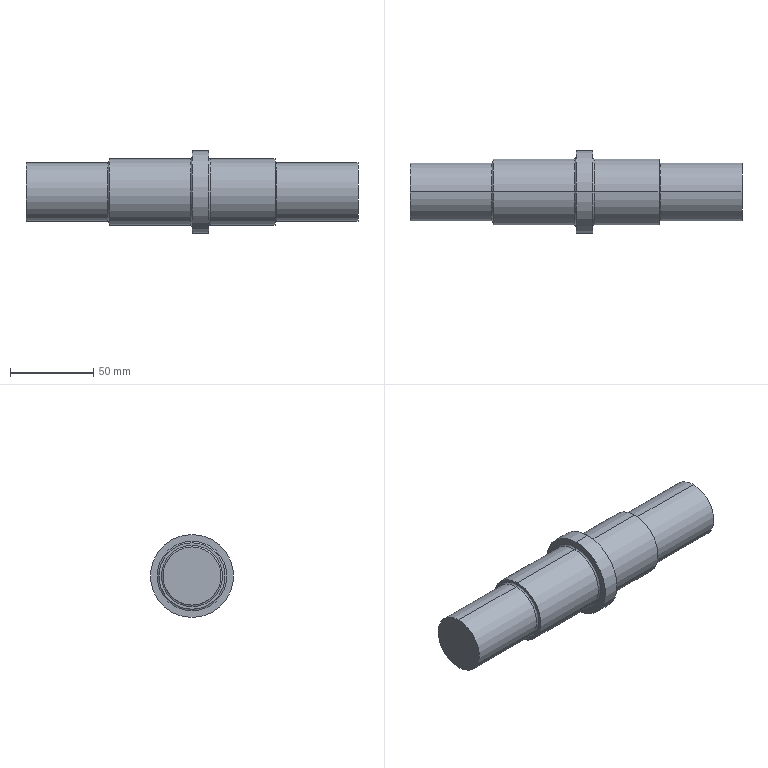Component | SolidWorks | AxisTwo-1 | 1 solid | 24 faces | box 200 x 50 x 50 mm | volume 229046 mm3 | cylinder 10 | torus 8 | plane 6 | commonest cylinder face diameters 35 x4 40 x4 50 x2
build123d program:
from build123d import *


with BuildPart() as part:
    # Sketch1 → Revolve1 (revolve)
    with BuildSketch(Plane(origin=(0, 0, 0), x_dir=(0, 0, -1), z_dir=(1, 0, 0)), mode=Mode.PRIVATE) as revolve1_sk:
        with BuildLine():
            Line((0, 0), (0, 17.5))
            Line((0, 17.5), (49, 17.5))
            ThreePointArc((49, 17.5), (49.707, 17.793), (50, 18.5))
            Line((50, 18.5), (50, 20))
            Line((50, 20), (89, 20))
            ThreePointArc((89, 20), (89.707, 20.293), (90, 21))
            Line((90, 21), (90, 25))
            Line((90, 25), (100, 25))
            Line((100, 25), (100, 21))
            ThreePointArc((100, 21), (100.293, 20.293), (101, 20))
            Line((101, 20), (150, 20))
            Line((150, 20), (150, 18.5))
            ThreePointArc((150, 18.5), (150.293, 17.793), (151, 17.5))
            Line((151, 17.5), (200, 17.5))
            Line((200, 17.5), (200, 0))
            Line((200, 0), (0, 0))
        make_face()
    revolve(revolve1_sk.sketch.rotate(Axis((0, 0, -200), (0, 0, 1)), 90), axis=Axis((0, 0, -200), (0, 0, 1)))


solid = part.part

# Placed as in the assembly
solid = solid.moved(Location((300.528, 15.31, -110), (0, 90, 0)))
STEP:
#1=COLOUR_RGB('',0.7922,0.8196,0.9333);
#2=FILL_AREA_STYLE_COLOUR('',#1);
#3=FILL_AREA_STYLE('',(#2));
#4=SURFACE_STYLE_FILL_AREA(#3);
#5=SURFACE_SIDE_STYLE('',(#4));
#6=SURFACE_STYLE_USAGE(.BOTH.,#5);
#7=PRESENTATION_STYLE_ASSIGNMENT((#6));
#8=CARTESIAN_POINT('',(11.832,0.6028,-3.642));
#9=VERTEX_POINT('',#8);
#10=CARTESIAN_POINT('',(11.832,0.6028,-5.02));
#11=VERTEX_POINT('',#10);
#12=CARTESIAN_POINT('',(11.832,0.6028,-4.331));
#13=DIRECTION('',(-1.,0.,0.));
#14=DIRECTION('',(0.,0.,1.));
#15=AXIS2_PLACEMENT_3D('',#12,#13,#14);
#16=CIRCLE('',#15,0.689);
#17=EDGE_CURVE('',#9,#11,#16,.T.);
#18=ORIENTED_EDGE('',*,*,#17,.T.);
#19=CARTESIAN_POINT('',(9.903,0.6028,-5.02));
#20=VERTEX_POINT('',#19);
#21=CARTESIAN_POINT('',(3.958,0.6028,-5.02));
#22=DIRECTION('',(-1.,0.,0.));
#23=VECTOR('',#22,39.37);
#24=LINE('',#21,#23);
#25=EDGE_CURVE('',#11,#20,#24,.T.);
#26=ORIENTED_EDGE('',*,*,#25,.T.);
#27=CARTESIAN_POINT('',(9.903,0.6028,-3.642));
#28=VERTEX_POINT('',#27);
#29=CARTESIAN_POINT('',(9.903,0.6028,-4.331));
#30=DIRECTION('',(-1.,0.,0.));
#31=DIRECTION('',(0.,0.,1.));
#32=AXIS2_PLACEMENT_3D('',#29,#30,#31);
#33=CIRCLE('',#32,0.689);
#34=EDGE_CURVE('',#28,#20,#33,.T.);
#35=ORIENTED_EDGE('',*,*,#34,.F.);
#36=CARTESIAN_POINT('',(3.958,0.6028,-3.642));
#37=DIRECTION('',(-1.,0.,0.));
#38=VECTOR('',#37,39.37);
#39=LINE('',#36,#38);
#40=EDGE_CURVE('',#9,#28,#39,.T.);
#41=ORIENTED_EDGE('',*,*,#40,.F.);
#42=EDGE_LOOP('',(#18,#26,#35,#41));
#43=FACE_OUTER_BOUND('',#42,.T.);
#44=CARTESIAN_POINT('',(3.958,0.6028,-4.331));
#45=DIRECTION('',(-1.,0.,0.));
#46=DIRECTION('',(0.,0.,1.));
#47=AXIS2_PLACEMENT_3D('',#44,#45,#46);
#48=CYLINDRICAL_SURFACE('',#47,0.689);
#49=ADVANCED_FACE('',(#43),#48,.T.);
#50=CARTESIAN_POINT('',(9.863,0.6028,-5.059));
#51=VERTEX_POINT('',#50);
#52=CARTESIAN_POINT('',(9.863,0.6028,-3.602));
#53=VERTEX_POINT('',#52);
#54=CARTESIAN_POINT('',(9.863,0.6028,-4.331));
#55=DIRECTION('',(-1.,0.,0.));
#56=DIRECTION('',(0.,0.,1.));
#57=AXIS2_PLACEMENT_3D('',#54,#55,#56);
#58=CIRCLE('',#57,0.7283);
#59=EDGE_CURVE('',#51,#53,#58,.T.);
#60=ORIENTED_EDGE('',*,*,#59,.F.);
#61=CARTESIAN_POINT('',(9.903,0.6028,-5.059));
#62=DIRECTION('',(0.,1.,0.));
#63=DIRECTION('',(0.,0.,1.));
#64=AXIS2_PLACEMENT_3D('',#61,#62,#63);
#65=CIRCLE('',#64,0.03937);
#66=EDGE_CURVE('',#51,#20,#65,.T.);
#67=ORIENTED_EDGE('',*,*,#66,.T.);
#68=CARTESIAN_POINT('',(9.903,0.6028,-4.331));
#69=DIRECTION('',(-1.,0.,0.));
#70=DIRECTION('',(0.,0.,1.));
#71=AXIS2_PLACEMENT_3D('',#68,#69,#70);
#72=CIRCLE('',#71,0.689);
#73=EDGE_CURVE('',#20,#28,#72,.T.);
#74=ORIENTED_EDGE('',*,*,#73,.T.);
#75=CARTESIAN_POINT('',(9.903,0.6028,-3.602));
#76=DIRECTION('',(0.,-1.,0.));
#77=DIRECTION('',(0.,0.,-1.));
#78=AXIS2_PLACEMENT_3D('',#75,#76,#77);
#79=CIRCLE('',#78,0.03937);
#80=EDGE_CURVE('',#53,#28,#79,.T.);
#81=ORIENTED_EDGE('',*,*,#80,.F.);
#82=EDGE_LOOP('',(#60,#67,#74,#81));
#83=FACE_OUTER_BOUND('',#82,.T.);
#84=CARTESIAN_POINT('',(9.903,0.6028,-4.331));
#85=DIRECTION('',(-1.,0.,0.));
#86=DIRECTION('',(0.,0.,1.));
#87=AXIS2_PLACEMENT_3D('',#84,#85,#86);
#88=TOROIDAL_SURFACE('',#87,0.7283,0.03937);
#89=ADVANCED_FACE('',(#83),#88,.F.);
#90=CARTESIAN_POINT('',(9.863,0.6028,-3.543));
#91=VERTEX_POINT('',#90);
#92=CARTESIAN_POINT('',(9.863,0.6028,-5.118));
#93=VERTEX_POINT('',#92);
#94=CARTESIAN_POINT('',(9.863,0.6028,-4.331));
#95=DIRECTION('',(-1.,0.,0.));
#96=DIRECTION('',(0.,0.,1.));
#97=AXIS2_PLACEMENT_3D('',#94,#95,#96);
#98=CIRCLE('',#97,0.7874);
#99=EDGE_CURVE('',#91,#93,#98,.T.);
#100=ORIENTED_EDGE('',*,*,#99,.T.);
#101=CARTESIAN_POINT('',(8.328,0.6028,-5.118));
#102=VERTEX_POINT('',#101);
#103=CARTESIAN_POINT('',(3.958,0.6028,-5.118));
#104=DIRECTION('',(-1.,0.,0.));
#105=VECTOR('',#104,39.37);
#106=LINE('',#103,#105);
#107=EDGE_CURVE('',#93,#102,#106,.T.);
#108=ORIENTED_EDGE('',*,*,#107,.T.);
#109=CARTESIAN_POINT('',(8.328,0.6028,-3.543));
#110=VERTEX_POINT('',#109);
#111=CARTESIAN_POINT('',(8.328,0.6028,-4.331));
#112=DIRECTION('',(-1.,0.,0.));
#113=DIRECTION('',(0.,0.,1.));
#114=AXIS2_PLACEMENT_3D('',#111,#112,#113);
#115=CIRCLE('',#114,0.7874);
#116=EDGE_CURVE('',#110,#102,#115,.T.);
#117=ORIENTED_EDGE('',*,*,#116,.F.);
#118=CARTESIAN_POINT('',(3.958,0.6028,-3.543));
#119=DIRECTION('',(-1.,0.,0.));
#120=VECTOR('',#119,39.37);
#121=LINE('',#118,#120);
#122=EDGE_CURVE('',#91,#110,#121,.T.);
#123=ORIENTED_EDGE('',*,*,#122,.F.);
#124=EDGE_LOOP('',(#100,#108,#117,#123));
#125=FACE_OUTER_BOUND('',#124,.T.);
#126=CARTESIAN_POINT('',(3.958,0.6028,-4.331));
#127=DIRECTION('',(-1.,0.,0.));
#128=DIRECTION('',(0.,0.,1.));
#129=AXIS2_PLACEMENT_3D('',#126,#127,#128);
#130=CYLINDRICAL_SURFACE('',#129,0.7874);
#131=ADVANCED_FACE('',(#125),#130,.T.);
#132=CARTESIAN_POINT('',(8.288,0.6028,-5.157));
#133=VERTEX_POINT('',#132);
#134=CARTESIAN_POINT('',(8.288,0.6028,-3.504));
#135=VERTEX_POINT('',#134);
#136=CARTESIAN_POINT('',(8.288,0.6028,-4.331));
#137=DIRECTION('',(-1.,0.,0.));
#138=DIRECTION('',(0.,0.,1.));
#139=AXIS2_PLACEMENT_3D('',#136,#137,#138);
#140=CIRCLE('',#139,0.8268);
#141=EDGE_CURVE('',#133,#135,#140,.T.);
#142=ORIENTED_EDGE('',*,*,#141,.F.);
#143=CARTESIAN_POINT('',(8.328,0.6028,-5.157));
#144=DIRECTION('',(0.,1.,0.));
#145=DIRECTION('',(0.,0.,1.));
#146=AXIS2_PLACEMENT_3D('',#143,#144,#145);
#147=CIRCLE('',#146,0.03937);
#148=EDGE_CURVE('',#133,#102,#147,.T.);
#149=ORIENTED_EDGE('',*,*,#148,.T.);
#150=CARTESIAN_POINT('',(8.328,0.6028,-4.331));
#151=DIRECTION('',(-1.,0.,0.));
#152=DIRECTION('',(0.,0.,1.));
#153=AXIS2_PLACEMENT_3D('',#150,#151,#152);
#154=CIRCLE('',#153,0.7874);
#155=EDGE_CURVE('',#102,#110,#154,.T.);
#156=ORIENTED_EDGE('',*,*,#155,.T.);
#157=CARTESIAN_POINT('',(8.328,0.6028,-3.504));
#158=DIRECTION('',(0.,-1.,0.));
#159=DIRECTION('',(0.,0.,-1.));
#160=AXIS2_PLACEMENT_3D('',#157,#158,#159);
#161=CIRCLE('',#160,0.03937);
#162=EDGE_CURVE('',#135,#110,#161,.T.);
#163=ORIENTED_EDGE('',*,*,#162,.F.);
#164=EDGE_LOOP('',(#142,#149,#156,#163));
#165=FACE_OUTER_BOUND('',#164,.T.);
#166=CARTESIAN_POINT('',(8.328,0.6028,-4.331));
#167=DIRECTION('',(-1.,0.,0.));
#168=DIRECTION('',(0.,0.,1.));
#169=AXIS2_PLACEMENT_3D('',#166,#167,#168);
#170=TOROIDAL_SURFACE('',#169,0.8268,0.03937);
#171=ADVANCED_FACE('',(#165),#170,.F.);
#172=CARTESIAN_POINT('',(8.288,0.6028,-3.346));
#173=VERTEX_POINT('',#172);
#174=CARTESIAN_POINT('',(8.288,0.6028,-5.315));
#175=VERTEX_POINT('',#174);
#176=CARTESIAN_POINT('',(8.288,0.6028,-4.331));
#177=DIRECTION('',(-1.,0.,0.));
#178=DIRECTION('',(0.,0.,1.));
#179=AXIS2_PLACEMENT_3D('',#176,#177,#178);
#180=CIRCLE('',#179,0.9843);
#181=EDGE_CURVE('',#173,#175,#180,.T.);
#182=ORIENTED_EDGE('',*,*,#181,.T.);
#183=CARTESIAN_POINT('',(7.895,0.6028,-5.315));
#184=VERTEX_POINT('',#183);
#185=CARTESIAN_POINT('',(3.958,0.6028,-5.315));
#186=DIRECTION('',(-1.,0.,0.));
#187=VECTOR('',#186,39.37);
#188=LINE('',#185,#187);
#189=EDGE_CURVE('',#175,#184,#188,.T.);
#190=ORIENTED_EDGE('',*,*,#189,.T.);
#191=CARTESIAN_POINT('',(7.895,0.6028,-3.346));
#192=VERTEX_POINT('',#191);
#193=CARTESIAN_POINT('',(7.895,0.6028,-4.331));
#194=DIRECTION('',(-1.,0.,0.));
#195=DIRECTION('',(0.,0.,1.));
#196=AXIS2_PLACEMENT_3D('',#193,#194,#195);
#197=CIRCLE('',#196,0.9843);
#198=EDGE_CURVE('',#192,#184,#197,.T.);
#199=ORIENTED_EDGE('',*,*,#198,.F.);
#200=CARTESIAN_POINT('',(3.958,0.6028,-3.346));
#201=DIRECTION('',(-1.,0.,0.));
#202=VECTOR('',#201,39.37);
#203=LINE('',#200,#202);
#204=EDGE_CURVE('',#173,#192,#203,.T.);
#205=ORIENTED_EDGE('',*,*,#204,.F.);
#206=EDGE_LOOP('',(#182,#190,#199,#205));
#207=FACE_OUTER_BOUND('',#206,.T.);
#208=CARTESIAN_POINT('',(3.958,0.6028,-4.331));
#209=DIRECTION('',(-1.,0.,0.));
#210=DIRECTION('',(0.,0.,1.));
#211=AXIS2_PLACEMENT_3D('',#208,#209,#210);
#212=CYLINDRICAL_SURFACE('',#211,0.9843);
#213=ADVANCED_FACE('',(#207),#212,.T.);
#214=CARTESIAN_POINT('',(7.855,0.6028,-5.118));
#215=VERTEX_POINT('',#214);
#216=CARTESIAN_POINT('',(7.855,0.6028,-3.543));
#217=VERTEX_POINT('',#216);
#218=CARTESIAN_POINT('',(7.855,0.6028,-4.331));
#219=DIRECTION('',(-1.,0.,0.));
#220=DIRECTION('',(0.,0.,1.));
#221=AXIS2_PLACEMENT_3D('',#218,#219,#220);
#222=CIRCLE('',#221,0.7874);
#223=EDGE_CURVE('',#215,#217,#222,.T.);
#224=ORIENTED_EDGE('',*,*,#223,.F.);
#225=CARTESIAN_POINT('',(7.895,0.6028,-5.157));
#226=VERTEX_POINT('',#225);
#227=CARTESIAN_POINT('',(7.855,0.6028,-5.157));
#228=DIRECTION('',(0.,1.,0.));
#229=DIRECTION('',(0.,0.,1.));
#230=AXIS2_PLACEMENT_3D('',#227,#228,#229);
#231=CIRCLE('',#230,0.03937);
#232=EDGE_CURVE('',#215,#226,#231,.T.);
#233=ORIENTED_EDGE('',*,*,#232,.T.);
#234=CARTESIAN_POINT('',(7.895,0.6028,-3.504));
#235=VERTEX_POINT('',#234);
#236=CARTESIAN_POINT('',(7.895,0.6028,-4.331));
#237=DIRECTION('',(-1.,0.,0.));
#238=DIRECTION('',(0.,0.,1.));
#239=AXIS2_PLACEMENT_3D('',#236,#237,#238);
#240=CIRCLE('',#239,0.8268);
#241=EDGE_CURVE('',#226,#235,#240,.T.);
#242=ORIENTED_EDGE('',*,*,#241,.T.);
#243=CARTESIAN_POINT('',(7.855,0.6028,-3.504));
#244=DIRECTION('',(0.,-1.,0.));
#245=DIRECTION('',(0.,0.,-1.));
#246=AXIS2_PLACEMENT_3D('',#243,#244,#245);
#247=CIRCLE('',#246,0.03937);
#248=EDGE_CURVE('',#217,#235,#247,.T.);
#249=ORIENTED_EDGE('',*,*,#248,.F.);
#250=EDGE_LOOP('',(#224,#233,#242,#249));
#251=FACE_OUTER_BOUND('',#250,.T.);
#252=CARTESIAN_POINT('',(7.855,0.6028,-4.331));
#253=DIRECTION('',(-1.,0.,0.));
#254=DIRECTION('',(0.,0.,1.));
#255=AXIS2_PLACEMENT_3D('',#252,#253,#254);
#256=TOROIDAL_SURFACE('',#255,0.8268,0.03937);
#257=ADVANCED_FACE('',(#251),#256,.F.);
#258=CARTESIAN_POINT('',(7.855,0.6028,-4.331));
#259=DIRECTION('',(-1.,0.,0.));
#260=DIRECTION('',(0.,0.,1.));
#261=AXIS2_PLACEMENT_3D('',#258,#259,#260);
#262=CIRCLE('',#261,0.7874);
#263=EDGE_CURVE('',#217,#215,#262,.T.);
#264=ORIENTED_EDGE('',*,*,#263,.T.);
#265=CARTESIAN_POINT('',(5.926,0.6028,-5.118));
#266=VERTEX_POINT('',#265);
#267=CARTESIAN_POINT('',(3.958,0.6028,-5.118));
#268=DIRECTION('',(-1.,0.,0.));
#269=VECTOR('',#268,39.37);
#270=LINE('',#267,#269);
#271=EDGE_CURVE('',#215,#266,#270,.T.);
#272=ORIENTED_EDGE('',*,*,#271,.T.);
#273=CARTESIAN_POINT('',(5.926,0.6028,-3.543));
#274=VERTEX_POINT('',#273);
#275=CARTESIAN_POINT('',(5.926,0.6028,-4.331));
#276=DIRECTION('',(-1.,0.,0.));
#277=DIRECTION('',(0.,0.,1.));
#278=AXIS2_PLACEMENT_3D('',#275,#276,#277);
#279=CIRCLE('',#278,0.7874);
#280=EDGE_CURVE('',#274,#266,#279,.T.);
#281=ORIENTED_EDGE('',*,*,#280,.F.);
#282=CARTESIAN_POINT('',(3.958,0.6028,-3.543));
#283=DIRECTION('',(-1.,0.,0.));
#284=VECTOR('',#283,39.37);
#285=LINE('',#282,#284);
#286=EDGE_CURVE('',#217,#274,#285,.T.);
#287=ORIENTED_EDGE('',*,*,#286,.F.);
#288=EDGE_LOOP('',(#264,#272,#281,#287));
#289=FACE_OUTER_BOUND('',#288,.T.);
#290=CARTESIAN_POINT('',(3.958,0.6028,-4.331));
#291=DIRECTION('',(-1.,0.,0.));
#292=DIRECTION('',(0.,0.,1.));
#293=AXIS2_PLACEMENT_3D('',#290,#291,#292);
#294=CYLINDRICAL_SURFACE('',#293,0.7874);
#295=ADVANCED_FACE('',(#289),#294,.T.);
#296=CARTESIAN_POINT('',(5.887,0.6028,-5.02));
#297=VERTEX_POINT('',#296);
#298=CARTESIAN_POINT('',(5.887,0.6028,-3.642));
#299=VERTEX_POINT('',#298);
#300=CARTESIAN_POINT('',(5.887,0.6028,-4.331));
#301=DIRECTION('',(-1.,0.,0.));
#302=DIRECTION('',(0.,0.,1.));
#303=AXIS2_PLACEMENT_3D('',#300,#301,#302);
#304=CIRCLE('',#303,0.689);
#305=EDGE_CURVE('',#297,#299,#304,.T.);
#306=ORIENTED_EDGE('',*,*,#305,.F.);
#307=CARTESIAN_POINT('',(5.926,0.6028,-5.059));
#308=VERTEX_POINT('',#307);
#309=CARTESIAN_POINT('',(5.887,0.6028,-5.059));
#310=DIRECTION('',(0.,1.,0.));
#311=DIRECTION('',(0.,0.,1.));
#312=AXIS2_PLACEMENT_3D('',#309,#310,#311);
#313=CIRCLE('',#312,0.03937);
#314=EDGE_CURVE('',#297,#308,#313,.T.);
#315=ORIENTED_EDGE('',*,*,#314,.T.);
#316=CARTESIAN_POINT('',(5.926,0.6028,-3.602));
#317=VERTEX_POINT('',#316);
#318=CARTESIAN_POINT('',(5.926,0.6028,-4.331));
#319=DIRECTION('',(-1.,0.,0.));
#320=DIRECTION('',(0.,0.,1.));
#321=AXIS2_PLACEMENT_3D('',#318,#319,#320);
#322=CIRCLE('',#321,0.7283);
#323=EDGE_CURVE('',#308,#317,#322,.T.);
#324=ORIENTED_EDGE('',*,*,#323,.T.);
#325=CARTESIAN_POINT('',(5.887,0.6028,-3.602));
#326=DIRECTION('',(0.,-1.,0.));
#327=DIRECTION('',(0.,0.,-1.));
#328=AXIS2_PLACEMENT_3D('',#325,#326,#327);
#329=CIRCLE('',#328,0.03937);
#330=EDGE_CURVE('',#299,#317,#329,.T.);
#331=ORIENTED_EDGE('',*,*,#330,.F.);
#332=EDGE_LOOP('',(#306,#315,#324,#331));
#333=FACE_OUTER_BOUND('',#332,.T.);
#334=CARTESIAN_POINT('',(5.887,0.6028,-4.331));
#335=DIRECTION('',(-1.,0.,0.));
#336=DIRECTION('',(0.,0.,1.));
#337=AXIS2_PLACEMENT_3D('',#334,#335,#336);
#338=TOROIDAL_SURFACE('',#337,0.7283,0.03937);
#339=ADVANCED_FACE('',(#333),#338,.F.);
#340=CARTESIAN_POINT('',(5.887,0.6028,-4.331));
#341=DIRECTION('',(-1.,0.,0.));
#342=DIRECTION('',(0.,0.,1.));
#343=AXIS2_PLACEMENT_3D('',#340,#341,#342);
#344=CIRCLE('',#343,0.689);
#345=EDGE_CURVE('',#299,#297,#344,.T.);
#346=ORIENTED_EDGE('',*,*,#345,.T.);
#347=CARTESIAN_POINT('',(3.958,0.6028,-5.02));
#348=VERTEX_POINT('',#347);
#349=CARTESIAN_POINT('',(3.958,0.6028,-5.02));
#350=DIRECTION('',(-1.,0.,0.));
#351=VECTOR('',#350,39.37);
#352=LINE('',#349,#351);
#353=EDGE_CURVE('',#297,#348,#352,.T.);
#354=ORIENTED_EDGE('',*,*,#353,.T.);
#355=CARTESIAN_POINT('',(3.958,0.6028,-3.642));
#356=VERTEX_POINT('',#355);
#357=CARTESIAN_POINT('',(3.958,0.6028,-4.331));
#358=DIRECTION('',(-1.,0.,0.));
#359=DIRECTION('',(0.,0.,1.));
#360=AXIS2_PLACEMENT_3D('',#357,#358,#359);
#361=CIRCLE('',#360,0.689);
#362=EDGE_CURVE('',#356,#348,#361,.T.);
#363=ORIENTED_EDGE('',*,*,#362,.F.);
#364=CARTESIAN_POINT('',(3.958,0.6028,-3.642));
#365=DIRECTION('',(-1.,0.,0.));
#366=VECTOR('',#365,39.37);
#367=LINE('',#364,#366);
#368=EDGE_CURVE('',#299,#356,#367,.T.);
#369=ORIENTED_EDGE('',*,*,#368,.F.);
#370=EDGE_LOOP('',(#346,#354,#363,#369));
#371=FACE_OUTER_BOUND('',#370,.T.);
#372=CARTESIAN_POINT('',(3.958,0.6028,-4.331));
#373=DIRECTION('',(-1.,0.,0.));
#374=DIRECTION('',(0.,0.,1.));
#375=AXIS2_PLACEMENT_3D('',#372,#373,#374);
#376=CYLINDRICAL_SURFACE('',#375,0.689);
#377=ADVANCED_FACE('',(#371),#376,.T.);
#378=ORIENTED_EDGE('',*,*,#362,.T.);
#379=CARTESIAN_POINT('',(3.958,0.6028,-4.331));
#380=DIRECTION('',(-1.,0.,0.));
#381=DIRECTION('',(0.,0.,1.));
#382=AXIS2_PLACEMENT_3D('',#379,#380,#381);
#383=CIRCLE('',#382,0.689);
#384=EDGE_CURVE('',#348,#356,#383,.T.);
#385=ORIENTED_EDGE('',*,*,#384,.T.);
#386=EDGE_LOOP('',(#378,#385));
#387=FACE_OUTER_BOUND('',#386,.T.);
#388=CARTESIAN_POINT('',(3.958,1.292,-4.331));
#389=DIRECTION('',(-1.,0.,0.));
#390=DIRECTION('',(0.,0.,1.));
#391=AXIS2_PLACEMENT_3D('',#388,#389,#390);
#392=PLANE('',#391);
#393=ADVANCED_FACE('',(#387),#392,.T.);
#394=ORIENTED_EDGE('',*,*,#353,.F.);
#395=ORIENTED_EDGE('',*,*,#305,.T.);
#396=ORIENTED_EDGE('',*,*,#368,.T.);
#397=ORIENTED_EDGE('',*,*,#384,.F.);
#398=EDGE_LOOP('',(#394,#395,#396,#397));
#399=FACE_OUTER_BOUND('',#398,.T.);
#400=CARTESIAN_POINT('',(3.958,0.6028,-4.331));
#401=DIRECTION('',(-1.,0.,0.));
#402=DIRECTION('',(0.,0.,1.));
#403=AXIS2_PLACEMENT_3D('',#400,#401,#402);
#404=CYLINDRICAL_SURFACE('',#403,0.689);
#405=ADVANCED_FACE('',(#399),#404,.T.);
#406=ORIENTED_EDGE('',*,*,#314,.F.);
#407=ORIENTED_EDGE('',*,*,#345,.F.);
#408=ORIENTED_EDGE('',*,*,#330,.T.);
#409=CARTESIAN_POINT('',(5.926,0.6028,-4.331));
#410=DIRECTION('',(-1.,0.,0.));
#411=DIRECTION('',(0.,0.,1.));
#412=AXIS2_PLACEMENT_3D('',#409,#410,#411);
#413=CIRCLE('',#412,0.7283);
#414=EDGE_CURVE('',#317,#308,#413,.T.);
#415=ORIENTED_EDGE('',*,*,#414,.T.);
#416=EDGE_LOOP('',(#406,#407,#408,#415));
#417=FACE_OUTER_BOUND('',#416,.T.);
#418=CARTESIAN_POINT('',(5.887,0.6028,-4.331));
#419=DIRECTION('',(-1.,0.,0.));
#420=DIRECTION('',(0.,0.,1.));
#421=AXIS2_PLACEMENT_3D('',#418,#419,#420);
#422=TOROIDAL_SURFACE('',#421,0.7283,0.03937);
#423=ADVANCED_FACE('',(#417),#422,.F.);
#424=ORIENTED_EDGE('',*,*,#280,.T.);
#425=CARTESIAN_POINT('',(5.926,0.6028,-4.331));
#426=DIRECTION('',(-1.,0.,0.));
#427=DIRECTION('',(0.,0.,1.));
#428=AXIS2_PLACEMENT_3D('',#425,#426,#427);
#429=CIRCLE('',#428,0.7874);
#430=EDGE_CURVE('',#266,#274,#429,.T.);
#431=ORIENTED_EDGE('',*,*,#430,.T.);
#432=EDGE_LOOP('',(#424,#431));
#433=FACE_OUTER_BOUND('',#432,.T.);
#434=ORIENTED_EDGE('',*,*,#414,.F.);
#435=ORIENTED_EDGE('',*,*,#323,.F.);
#436=EDGE_LOOP('',(#434,#435));
#437=FACE_BOUND('',#436,.T.);
#438=CARTESIAN_POINT('',(5.926,1.39,-4.331));
#439=DIRECTION('',(-1.,0.,0.));
#440=DIRECTION('',(0.,0.,1.));
#441=AXIS2_PLACEMENT_3D('',#438,#439,#440);
#442=PLANE('',#441);
#443=ADVANCED_FACE('',(#433,#437),#442,.T.);
#444=ORIENTED_EDGE('',*,*,#271,.F.);
#445=ORIENTED_EDGE('',*,*,#223,.T.);
#446=ORIENTED_EDGE('',*,*,#286,.T.);
#447=ORIENTED_EDGE('',*,*,#430,.F.);
#448=EDGE_LOOP('',(#444,#445,#446,#447));
#449=FACE_OUTER_BOUND('',#448,.T.);
#450=CARTESIAN_POINT('',(3.958,0.6028,-4.331));
#451=DIRECTION('',(-1.,0.,0.));
#452=DIRECTION('',(0.,0.,1.));
#453=AXIS2_PLACEMENT_3D('',#450,#451,#452);
#454=CYLINDRICAL_SURFACE('',#453,0.7874);
#455=ADVANCED_FACE('',(#449),#454,.T.);
#456=ORIENTED_EDGE('',*,*,#232,.F.);
#457=ORIENTED_EDGE('',*,*,#263,.F.);
#458=ORIENTED_EDGE('',*,*,#248,.T.);
#459=CARTESIAN_POINT('',(7.895,0.6028,-4.331));
#460=DIRECTION('',(-1.,0.,0.));
#461=DIRECTION('',(0.,0.,1.));
#462=AXIS2_PLACEMENT_3D('',#459,#460,#461);
#463=CIRCLE('',#462,0.8268);
#464=EDGE_CURVE('',#235,#226,#463,.T.);
#465=ORIENTED_EDGE('',*,*,#464,.T.);
#466=EDGE_LOOP('',(#456,#457,#458,#465));
#467=FACE_OUTER_BOUND('',#466,.T.);
#468=CARTESIAN_POINT('',(7.855,0.6028,-4.331));
#469=DIRECTION('',(-1.,0.,0.));
#470=DIRECTION('',(0.,0.,1.));
#471=AXIS2_PLACEMENT_3D('',#468,#469,#470);
#472=TOROIDAL_SURFACE('',#471,0.8268,0.03937);
#473=ADVANCED_FACE('',(#467),#472,.F.);
#474=ORIENTED_EDGE('',*,*,#198,.T.);
#475=CARTESIAN_POINT('',(7.895,0.6028,-4.331));
#476=DIRECTION('',(-1.,0.,0.));
#477=DIRECTION('',(0.,0.,1.));
#478=AXIS2_PLACEMENT_3D('',#475,#476,#477);
#479=CIRCLE('',#478,0.9843);
#480=EDGE_CURVE('',#184,#192,#479,.T.);
#481=ORIENTED_EDGE('',*,*,#480,.T.);
#482=EDGE_LOOP('',(#474,#481));
#483=FACE_OUTER_BOUND('',#482,.T.);
#484=ORIENTED_EDGE('',*,*,#464,.F.);
#485=ORIENTED_EDGE('',*,*,#241,.F.);
#486=EDGE_LOOP('',(#484,#485));
#487=FACE_BOUND('',#486,.T.);
#488=CARTESIAN_POINT('',(7.895,1.587,-4.331));
#489=DIRECTION('',(-1.,0.,0.));
#490=DIRECTION('',(0.,0.,1.));
#491=AXIS2_PLACEMENT_3D('',#488,#489,#490);
#492=PLANE('',#491);
#493=ADVANCED_FACE('',(#483,#487),#492,.T.);
#494=ORIENTED_EDGE('',*,*,#189,.F.);
#495=CARTESIAN_POINT('',(8.288,0.6028,-4.331));
#496=DIRECTION('',(-1.,0.,0.));
#497=DIRECTION('',(0.,0.,1.));
#498=AXIS2_PLACEMENT_3D('',#495,#496,#497);
#499=CIRCLE('',#498,0.9843);
#500=EDGE_CURVE('',#175,#173,#499,.T.);
#501=ORIENTED_EDGE('',*,*,#500,.T.);
#502=ORIENTED_EDGE('',*,*,#204,.T.);
#503=ORIENTED_EDGE('',*,*,#480,.F.);
#504=EDGE_LOOP('',(#494,#501,#502,#503));
#505=FACE_OUTER_BOUND('',#504,.T.);
#506=CARTESIAN_POINT('',(3.958,0.6028,-4.331));
#507=DIRECTION('',(-1.,0.,0.));
#508=DIRECTION('',(0.,0.,1.));
#509=AXIS2_PLACEMENT_3D('',#506,#507,#508);
#510=CYLINDRICAL_SURFACE('',#509,0.9843);
#511=ADVANCED_FACE('',(#505),#510,.T.);
#512=CARTESIAN_POINT('',(8.288,0.6028,-4.331));
#513=DIRECTION('',(-1.,0.,0.));
#514=DIRECTION('',(0.,0.,1.));
#515=AXIS2_PLACEMENT_3D('',#512,#513,#514);
#516=CIRCLE('',#515,0.8268);
#517=EDGE_CURVE('',#135,#133,#516,.T.);
#518=ORIENTED_EDGE('',*,*,#517,.T.);
#519=ORIENTED_EDGE('',*,*,#141,.T.);
#520=EDGE_LOOP('',(#518,#519));
#521=FACE_BOUND('',#520,.T.);
#522=ORIENTED_EDGE('',*,*,#181,.F.);
#523=ORIENTED_EDGE('',*,*,#500,.F.);
#524=EDGE_LOOP('',(#522,#523));
#525=FACE_OUTER_BOUND('',#524,.T.);
#526=CARTESIAN_POINT('',(8.288,1.43,-4.331));
#527=DIRECTION('',(1.,0.,0.));
#528=DIRECTION('',(0.,0.,-1.));
#529=AXIS2_PLACEMENT_3D('',#526,#527,#528);
#530=PLANE('',#529);
#531=ADVANCED_FACE('',(#521,#525),#530,.T.);
#532=ORIENTED_EDGE('',*,*,#148,.F.);
#533=ORIENTED_EDGE('',*,*,#517,.F.);
#534=ORIENTED_EDGE('',*,*,#162,.T.);
#535=ORIENTED_EDGE('',*,*,#116,.T.);
#536=EDGE_LOOP('',(#532,#533,#534,#535));
#537=FACE_OUTER_BOUND('',#536,.T.);
#538=CARTESIAN_POINT('',(8.328,0.6028,-4.331));
#539=DIRECTION('',(-1.,0.,0.));
#540=DIRECTION('',(0.,0.,1.));
#541=AXIS2_PLACEMENT_3D('',#538,#539,#540);
#542=TOROIDAL_SURFACE('',#541,0.8268,0.03937);
#543=ADVANCED_FACE('',(#537),#542,.F.);
#544=ORIENTED_EDGE('',*,*,#107,.F.);
#545=CARTESIAN_POINT('',(9.863,0.6028,-4.331));
#546=DIRECTION('',(-1.,0.,0.));
#547=DIRECTION('',(0.,0.,1.));
#548=AXIS2_PLACEMENT_3D('',#545,#546,#547);
#549=CIRCLE('',#548,0.7874);
#550=EDGE_CURVE('',#93,#91,#549,.T.);
#551=ORIENTED_EDGE('',*,*,#550,.T.);
#552=ORIENTED_EDGE('',*,*,#122,.T.);
#553=ORIENTED_EDGE('',*,*,#155,.F.);
#554=EDGE_LOOP('',(#544,#551,#552,#553));
#555=FACE_OUTER_BOUND('',#554,.T.);
#556=CARTESIAN_POINT('',(3.958,0.6028,-4.331));
#557=DIRECTION('',(-1.,0.,0.));
#558=DIRECTION('',(0.,0.,1.));
#559=AXIS2_PLACEMENT_3D('',#556,#557,#558);
#560=CYLINDRICAL_SURFACE('',#559,0.7874);
#561=ADVANCED_FACE('',(#555),#560,.T.);
#562=CARTESIAN_POINT('',(9.863,0.6028,-4.331));
#563=DIRECTION('',(-1.,0.,0.));
#564=DIRECTION('',(0.,0.,1.));
#565=AXIS2_PLACEMENT_3D('',#562,#563,#564);
#566=CIRCLE('',#565,0.7283);
#567=EDGE_CURVE('',#53,#51,#566,.T.);
#568=ORIENTED_EDGE('',*,*,#567,.T.);
#569=ORIENTED_EDGE('',*,*,#59,.T.);
#570=EDGE_LOOP('',(#568,#569));
#571=FACE_BOUND('',#570,.T.);
#572=ORIENTED_EDGE('',*,*,#99,.F.);
#573=ORIENTED_EDGE('',*,*,#550,.F.);
#574=EDGE_LOOP('',(#572,#573));
#575=FACE_OUTER_BOUND('',#574,.T.);
#576=CARTESIAN_POINT('',(9.863,1.331,-4.331));
#577=DIRECTION('',(1.,0.,0.));
#578=DIRECTION('',(0.,0.,-1.));
#579=AXIS2_PLACEMENT_3D('',#576,#577,#578);
#580=PLANE('',#579);
#581=ADVANCED_FACE('',(#571,#575),#580,.T.);
#582=ORIENTED_EDGE('',*,*,#66,.F.);
#583=ORIENTED_EDGE('',*,*,#567,.F.);
#584=ORIENTED_EDGE('',*,*,#80,.T.);
#585=ORIENTED_EDGE('',*,*,#34,.T.);
#586=EDGE_LOOP('',(#582,#583,#584,#585));
#587=FACE_OUTER_BOUND('',#586,.T.);
#588=CARTESIAN_POINT('',(9.903,0.6028,-4.331));
#589=DIRECTION('',(-1.,0.,0.));
#590=DIRECTION('',(0.,0.,1.));
#591=AXIS2_PLACEMENT_3D('',#588,#589,#590);
#592=TOROIDAL_SURFACE('',#591,0.7283,0.03937);
#593=ADVANCED_FACE('',(#587),#592,.F.);
#594=ORIENTED_EDGE('',*,*,#25,.F.);
#595=CARTESIAN_POINT('',(11.832,0.6028,-4.331));
#596=DIRECTION('',(-1.,0.,0.));
#597=DIRECTION('',(0.,0.,1.));
#598=AXIS2_PLACEMENT_3D('',#595,#596,#597);
#599=CIRCLE('',#598,0.689);
#600=EDGE_CURVE('',#11,#9,#599,.T.);
#601=ORIENTED_EDGE('',*,*,#600,.T.);
#602=ORIENTED_EDGE('',*,*,#40,.T.);
#603=ORIENTED_EDGE('',*,*,#73,.F.);
#604=EDGE_LOOP('',(#594,#601,#602,#603));
#605=FACE_OUTER_BOUND('',#604,.T.);
#606=CARTESIAN_POINT('',(3.958,0.6028,-4.331));
#607=DIRECTION('',(-1.,0.,0.));
#608=DIRECTION('',(0.,0.,1.));
#609=AXIS2_PLACEMENT_3D('',#606,#607,#608);
#610=CYLINDRICAL_SURFACE('',#609,0.689);
#611=ADVANCED_FACE('',(#605),#610,.T.);
#612=ORIENTED_EDGE('',*,*,#17,.F.);
#613=ORIENTED_EDGE('',*,*,#600,.F.);
#614=EDGE_LOOP('',(#612,#613));
#615=FACE_OUTER_BOUND('',#614,.T.);
#616=CARTESIAN_POINT('',(11.832,0.6028,-4.331));
#617=DIRECTION('',(1.,0.,0.));
#618=DIRECTION('',(0.,0.,-1.));
#619=AXIS2_PLACEMENT_3D('',#616,#617,#618);
#620=PLANE('',#619);
#621=ADVANCED_FACE('',(#615),#620,.T.);
#622=CLOSED_SHELL('',(#49,#89,#131,#171,#213,#257,#295,#339,#377,#393,#405,#423,#443,#455,#473,#493,#511,#531,#543,#561,#581,#593,#611,#621));
#623=MANIFOLD_SOLID_BREP('',#622);
#624=STYLED_ITEM('',(#7),#623);
#625=PRESENTATION_LAYER_ASSIGNMENT('','',(#624));
#626=(LENGTH_UNIT()NAMED_UNIT(*)SI_UNIT($,.METRE.));
#627=LENGTH_MEASURE_WITH_UNIT(LENGTH_MEASURE(0.0254),#626);
#628=DIMENSIONAL_EXPONENTS(1.,0.,0.,0.,0.,0.,0.);
#629=(CONVERSION_BASED_UNIT('',#627)LENGTH_UNIT()NAMED_UNIT(#628));
#630=UNCERTAINTY_MEASURE_WITH_UNIT(LENGTH_MEASURE(0.00001),#629,'','');
#631=(NAMED_UNIT(*)PLANE_ANGLE_UNIT()SI_UNIT($,.RADIAN.));
#632=(NAMED_UNIT(*)SI_UNIT($,.STERADIAN.)SOLID_ANGLE_UNIT());
#633=(GEOMETRIC_REPRESENTATION_CONTEXT(3)GLOBAL_UNCERTAINTY_ASSIGNED_CONTEXT((#630))GLOBAL_UNIT_ASSIGNED_CONTEXT((#629,#631,#632))REPRESENTATION_CONTEXT('',''));
#634=MECHANICAL_DESIGN_GEOMETRIC_PRESENTATION_REPRESENTATION('',(#624),#633);
#635=CARTESIAN_POINT('',(0.,0.,0.));
#636=DIRECTION('',(0.,0.,1.));
#637=DIRECTION('',(1.,0.,0.));
#638=AXIS2_PLACEMENT_3D('',#635,#636,#637);
#639=(LENGTH_UNIT()NAMED_UNIT(*)SI_UNIT($,.METRE.));
#640=LENGTH_MEASURE_WITH_UNIT(LENGTH_MEASURE(0.0254),#639);
#641=DIMENSIONAL_EXPONENTS(1.,0.,0.,0.,0.,0.,0.);
#642=(CONVERSION_BASED_UNIT('',#640)LENGTH_UNIT()NAMED_UNIT(#641));
#643=UNCERTAINTY_MEASURE_WITH_UNIT(LENGTH_MEASURE(0.00001),#642,'','');
#644=(NAMED_UNIT(*)PLANE_ANGLE_UNIT()SI_UNIT($,.RADIAN.));
#645=(NAMED_UNIT(*)SI_UNIT($,.STERADIAN.)SOLID_ANGLE_UNIT());
#646=(GEOMETRIC_REPRESENTATION_CONTEXT(3)GLOBAL_UNCERTAINTY_ASSIGNED_CONTEXT((#643))GLOBAL_UNIT_ASSIGNED_CONTEXT((#642,#644,#645))REPRESENTATION_CONTEXT('',''));
#647=ADVANCED_BREP_SHAPE_REPRESENTATION('',(#623,#638),#646);